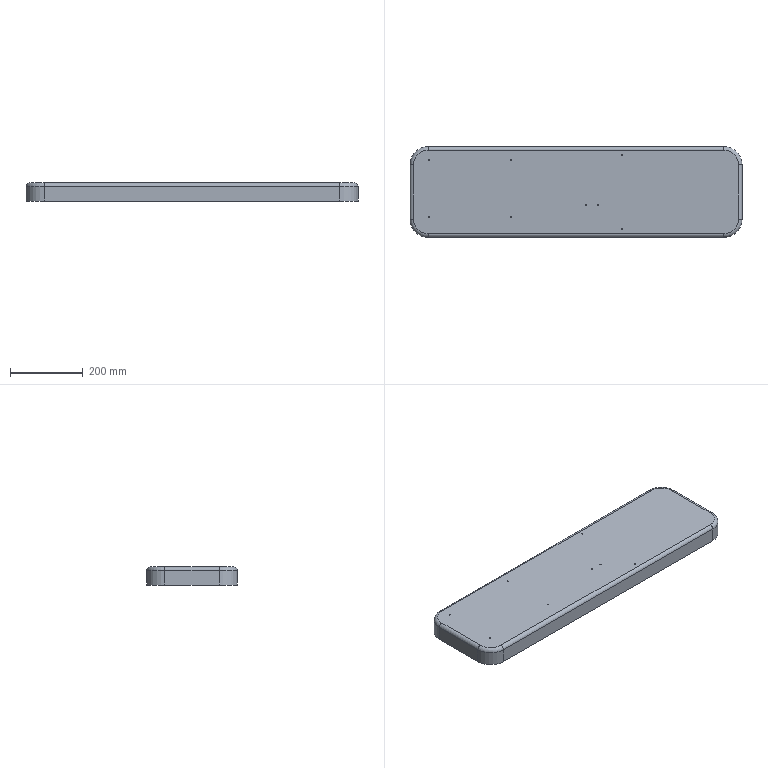Component | NX | BASE | 1 solid | 26 faces | volume 11279513 mm3 | cylinder 16 | plane 6 | torus 4 | commonest cylinder face diameters 3 x8 100 x4 20 x4